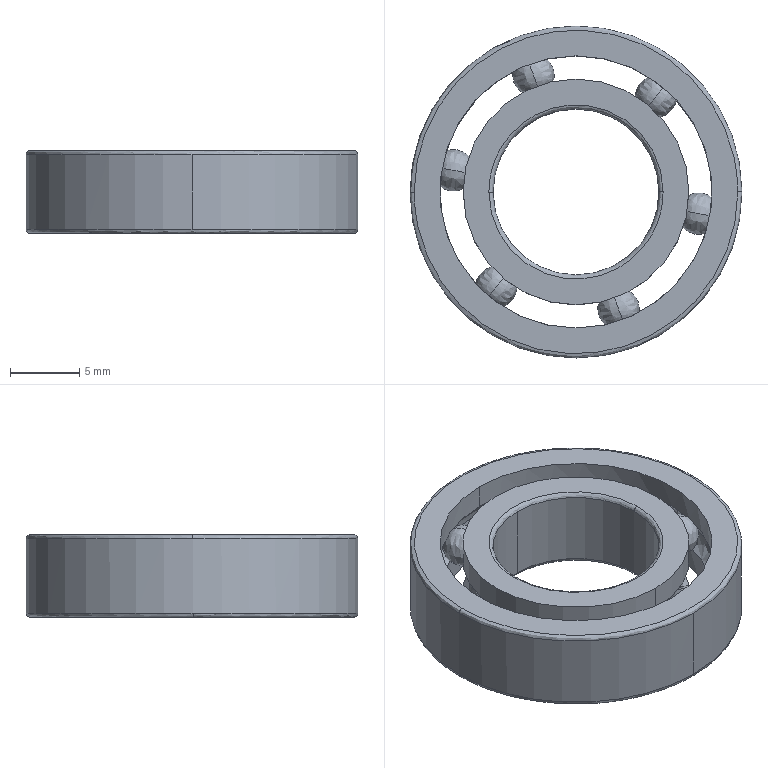Component | SolidWorks | 61901Bearing-2 | 8 solids | 42 faces | volume 1416 mm3 | spline 26 | cylinder 12 | plane 4 | commonest cylinder face diameters 16.32 x4 19.68 x4 12 x2 24 x2 | material 45#Steel